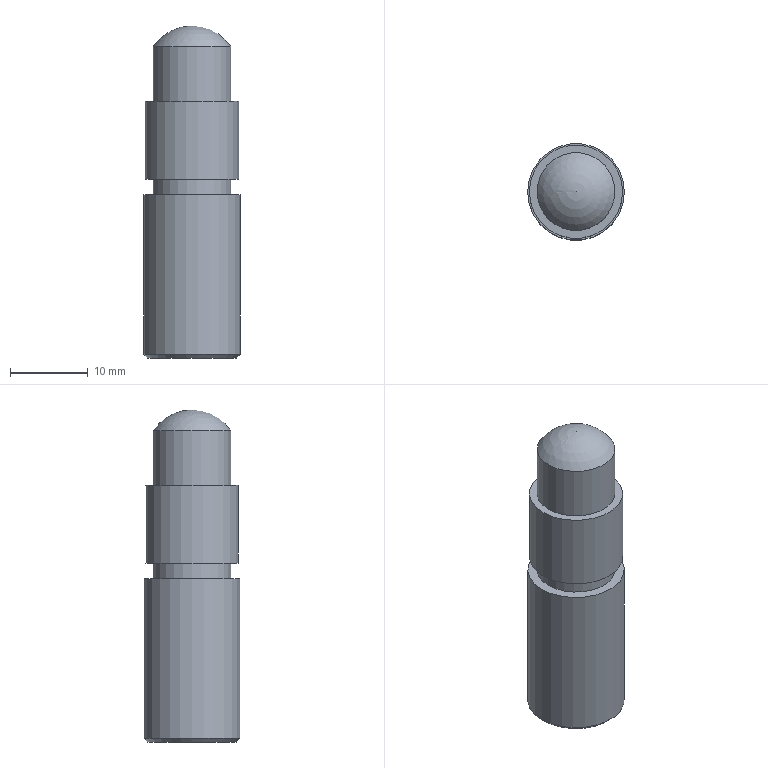Component | NX | EJECTOR_PIN | 1 solid | 10 faces | box 12.42 x 12.42 x 42.68 mm | volume 4494 mm3 | plane 4 | cylinder 4 | sphere 1 | cone 1 | commonest cylinder face diameters 10 x2 12.423 x1 12 x1
STEP:
#1=CARTESIAN_POINT('',(0.,0.,0.));
#2=DIRECTION('',(0.,0.,1.));
#3=DIRECTION('',(1.,0.,0.));
#4=AXIS2_PLACEMENT_3D('',#1,#2,#3);
#5=CARTESIAN_POINT('',(12.5,-0.,99.003));
#6=VERTEX_POINT('',#5);
#7=CARTESIAN_POINT('',(7.5,-0.,99.003));
#8=DIRECTION('',(0.,0.,1.));
#9=DIRECTION('',(1.,0.,0.));
#10=AXIS2_PLACEMENT_3D('',#7,#8,#9);
#11=CIRCLE('',#10,5.);
#12=CARTESIAN_POINT('',(7.5,-0.,99.003));
#13=DIRECTION('',(0.,0.,1.));
#14=DIRECTION('',(1.,0.,0.));
#15=AXIS2_PLACEMENT_3D('',#12,#13,#14);
#16=PLANE('',#15);
#17=CARTESIAN_POINT('',(0.,-0.));
#18=DIRECTION('',(1.,0.));
#19=AXIS2_PLACEMENT_2D('',#17,#18);
#20=CIRCLE('',#19,5.);
#21=(GEOMETRIC_REPRESENTATION_CONTEXT(2)PARAMETRIC_REPRESENTATION_CONTEXT()REPRESENTATION_CONTEXT('',''));
#22=DEFINITIONAL_REPRESENTATION('',(#20),#21);
#23=PCURVE('',#16,#22);
#24=CARTESIAN_POINT('',(7.5,-0.,99.003));
#25=DIRECTION('',(0.,0.,1.));
#26=DIRECTION('',(1.,0.,0.));
#27=AXIS2_PLACEMENT_3D('',#24,#25,#26);
#28=CYLINDRICAL_SURFACE('',#27,5.);
#29=CARTESIAN_POINT('',(0.,0.));
#30=DIRECTION('',(1.,0.));
#31=VECTOR('',#30,1.);
#32=LINE('',#29,#31);
#33=(GEOMETRIC_REPRESENTATION_CONTEXT(2)PARAMETRIC_REPRESENTATION_CONTEXT()REPRESENTATION_CONTEXT('',''));
#34=DEFINITIONAL_REPRESENTATION('',(#32),#33);
#35=PCURVE('',#28,#34);
#36=SURFACE_CURVE('',#11,(#23,#35),.PCURVE_S1.);
#37=EDGE_CURVE('',#6,#6,#36,.T.);
#38=ORIENTED_EDGE('',*,*,#37,.F.);
#39=EDGE_LOOP('',(#38));
#40=FACE_BOUND('',#39,.T.);
#41=CARTESIAN_POINT('',(13.712,-0.,99.003));
#42=VERTEX_POINT('',#41);
#43=CARTESIAN_POINT('',(7.5,-0.,99.003));
#44=DIRECTION('',(0.,0.,-1.));
#45=DIRECTION('',(1.,0.,0.));
#46=AXIS2_PLACEMENT_3D('',#43,#44,#45);
#47=CIRCLE('',#46,6.212);
#48=CARTESIAN_POINT('',(6.212,0.));
#49=CARTESIAN_POINT('',(6.212,-10.759));
#50=CARTESIAN_POINT('',(-3.106,-5.379));
#51=CARTESIAN_POINT('',(-12.423,-0.));
#52=CARTESIAN_POINT('',(-3.106,5.379));
#53=CARTESIAN_POINT('',(6.212,10.759));
#54=CARTESIAN_POINT('',(6.212,0.));
#55=(BOUNDED_CURVE()B_SPLINE_CURVE(2,(#48,#49,#50,#51,#52,#53,#54),.UNSPECIFIED.,.T.,.F.)B_SPLINE_CURVE_WITH_KNOTS((1,2,2,2,2,1),(-2.094,0.,2.094,4.189,6.283,8.378),.UNSPECIFIED.)CURVE()GEOMETRIC_REPRESENTATION_ITEM()RATIONAL_B_SPLINE_CURVE((1.,0.5,1.,0.5,1.,0.5,1.))REPRESENTATION_ITEM(''));
#56=(GEOMETRIC_REPRESENTATION_CONTEXT(2)PARAMETRIC_REPRESENTATION_CONTEXT()REPRESENTATION_CONTEXT('',''));
#57=DEFINITIONAL_REPRESENTATION('',(#55),#56);
#58=PCURVE('',#16,#57);
#59=CARTESIAN_POINT('',(7.5,-0.,78.003));
#60=DIRECTION('',(0.,0.,1.));
#61=DIRECTION('',(1.,0.,0.));
#62=AXIS2_PLACEMENT_3D('',#59,#60,#61);
#63=CYLINDRICAL_SURFACE('',#62,6.212);
#64=CARTESIAN_POINT('',(6.283,21.));
#65=DIRECTION('',(-1.,0.));
#66=VECTOR('',#65,1.);
#67=LINE('',#64,#66);
#68=(GEOMETRIC_REPRESENTATION_CONTEXT(2)PARAMETRIC_REPRESENTATION_CONTEXT()REPRESENTATION_CONTEXT('',''));
#69=DEFINITIONAL_REPRESENTATION('',(#67),#68);
#70=PCURVE('',#63,#69);
#71=SURFACE_CURVE('',#47,(#58,#70),.PCURVE_S1.);
#72=EDGE_CURVE('',#42,#42,#71,.T.);
#73=ORIENTED_EDGE('',*,*,#72,.F.);
#74=EDGE_LOOP('',(#73));
#75=FACE_BOUND('',#74,.T.);
#76=ADVANCED_FACE('',(#40,#75),#16,.T.);
#77=CARTESIAN_POINT('',(1.788,-0.,78.003));
#78=VERTEX_POINT('',#77);
#79=CARTESIAN_POINT('',(7.5,-0.,78.003));
#80=DIRECTION('',(0.,0.,-1.));
#81=DIRECTION('',(-1.,0.,0.));
#82=AXIS2_PLACEMENT_3D('',#79,#80,#81);
#83=CIRCLE('',#82,5.712);
#84=CARTESIAN_POINT('',(7.5,-0.,78.003));
#85=DIRECTION('',(0.,0.,-1.));
#86=DIRECTION('',(-1.,0.,0.));
#87=AXIS2_PLACEMENT_3D('',#84,#85,#86);
#88=PLANE('',#87);
#89=CARTESIAN_POINT('',(0.,0.));
#90=DIRECTION('',(1.,0.));
#91=AXIS2_PLACEMENT_2D('',#89,#90);
#92=CIRCLE('',#91,5.712);
#93=(GEOMETRIC_REPRESENTATION_CONTEXT(2)PARAMETRIC_REPRESENTATION_CONTEXT()REPRESENTATION_CONTEXT('',''));
#94=DEFINITIONAL_REPRESENTATION('',(#92),#93);
#95=PCURVE('',#88,#94);
#96=CARTESIAN_POINT('',(7.5,-0.,78.503));
#97=DIRECTION('',(0.,0.,1.));
#98=DIRECTION('',(1.,0.,0.));
#99=AXIS2_PLACEMENT_3D('',#96,#97,#98);
#100=CONICAL_SURFACE('',#99,6.212,0.7854);
#101=CARTESIAN_POINT('',(9.425,-0.5));
#102=DIRECTION('',(-1.,0.));
#103=VECTOR('',#102,1.);
#104=LINE('',#101,#103);
#105=(GEOMETRIC_REPRESENTATION_CONTEXT(2)PARAMETRIC_REPRESENTATION_CONTEXT()REPRESENTATION_CONTEXT('',''));
#106=DEFINITIONAL_REPRESENTATION('',(#104),#105);
#107=PCURVE('',#100,#106);
#108=SURFACE_CURVE('',#83,(#95,#107),.PCURVE_S1.);
#109=EDGE_CURVE('',#78,#78,#108,.T.);
#110=ORIENTED_EDGE('',*,*,#109,.T.);
#111=EDGE_LOOP('',(#110));
#112=FACE_BOUND('',#111,.T.);
#113=ADVANCED_FACE('',(#112),#88,.T.);
#114=CARTESIAN_POINT('',(1.288,-0.,78.503));
#115=VERTEX_POINT('',#114);
#116=CARTESIAN_POINT('',(13.712,-0.,78.503));
#117=VERTEX_POINT('',#116);
#118=CARTESIAN_POINT('',(7.5,-0.,78.503));
#119=DIRECTION('',(0.,0.,1.));
#120=DIRECTION('',(-1.,0.,0.));
#121=AXIS2_PLACEMENT_3D('',#118,#119,#120);
#122=CIRCLE('',#121,6.212);
#123=CARTESIAN_POINT('',(3.142,0.5));
#124=DIRECTION('',(1.,0.));
#125=VECTOR('',#124,1.);
#126=LINE('',#123,#125);
#127=(GEOMETRIC_REPRESENTATION_CONTEXT(2)PARAMETRIC_REPRESENTATION_CONTEXT()REPRESENTATION_CONTEXT('',''));
#128=DEFINITIONAL_REPRESENTATION('',(#126),#127);
#129=PCURVE('',#63,#128);
#130=CARTESIAN_POINT('',(3.142,0.));
#131=DIRECTION('',(1.,-0.));
#132=VECTOR('',#131,1.);
#133=LINE('',#130,#132);
#134=(GEOMETRIC_REPRESENTATION_CONTEXT(2)PARAMETRIC_REPRESENTATION_CONTEXT()REPRESENTATION_CONTEXT('',''));
#135=DEFINITIONAL_REPRESENTATION('',(#133),#134);
#136=PCURVE('',#100,#135);
#137=SURFACE_CURVE('',#122,(#129,#136),.PCURVE_S1.);
#138=EDGE_CURVE('',#115,#117,#137,.T.);
#139=ORIENTED_EDGE('',*,*,#138,.T.);
#140=CARTESIAN_POINT('',(13.712,-0.,78.503));
#141=CARTESIAN_POINT('',(13.712,-0.,99.003));
#142=B_SPLINE_CURVE_WITH_KNOTS('',1,(#140,#141),.UNSPECIFIED.,.F.,.F.,(2,2),(0.5,21.),.PIECEWISE_BEZIER_KNOTS.);
#143=CARTESIAN_POINT('',(6.283,0.));
#144=DIRECTION('',(0.,1.));
#145=VECTOR('',#144,1.);
#146=LINE('',#143,#145);
#147=(GEOMETRIC_REPRESENTATION_CONTEXT(2)PARAMETRIC_REPRESENTATION_CONTEXT()REPRESENTATION_CONTEXT('',''));
#148=DEFINITIONAL_REPRESENTATION('',(#146),#147);
#149=PCURVE('',#63,#148);
#150=CARTESIAN_POINT('',(0.,0.));
#151=DIRECTION('',(0.,1.));
#152=VECTOR('',#151,1.);
#153=LINE('',#150,#152);
#154=(GEOMETRIC_REPRESENTATION_CONTEXT(2)PARAMETRIC_REPRESENTATION_CONTEXT()REPRESENTATION_CONTEXT('',''));
#155=DEFINITIONAL_REPRESENTATION('',(#153),#154);
#156=PCURVE('',#63,#155);
#157=SEAM_CURVE('',#142,(#149,#156),.PCURVE_S1.);
#158=EDGE_CURVE('',#117,#42,#157,.T.);
#159=ORIENTED_EDGE('',*,*,#158,.T.);
#160=ORIENTED_EDGE('',*,*,#72,.T.);
#161=ORIENTED_EDGE('',*,*,#158,.F.);
#162=CARTESIAN_POINT('',(7.5,-0.,78.503));
#163=DIRECTION('',(0.,0.,1.));
#164=DIRECTION('',(-1.,0.,0.));
#165=AXIS2_PLACEMENT_3D('',#162,#163,#164);
#166=CIRCLE('',#165,6.212);
#167=CARTESIAN_POINT('',(-3.142,0.5));
#168=DIRECTION('',(1.,0.));
#169=VECTOR('',#168,1.);
#170=LINE('',#167,#169);
#171=(GEOMETRIC_REPRESENTATION_CONTEXT(2)PARAMETRIC_REPRESENTATION_CONTEXT()REPRESENTATION_CONTEXT('',''));
#172=DEFINITIONAL_REPRESENTATION('',(#170),#171);
#173=PCURVE('',#63,#172);
#174=CARTESIAN_POINT('',(3.142,-0.));
#175=DIRECTION('',(1.,0.));
#176=VECTOR('',#175,1.);
#177=LINE('',#174,#176);
#178=(GEOMETRIC_REPRESENTATION_CONTEXT(2)PARAMETRIC_REPRESENTATION_CONTEXT()REPRESENTATION_CONTEXT('',''));
#179=DEFINITIONAL_REPRESENTATION('',(#177),#178);
#180=PCURVE('',#100,#179);
#181=SURFACE_CURVE('',#166,(#173,#180),.PCURVE_S1.);
#182=EDGE_CURVE('',#117,#115,#181,.T.);
#183=ORIENTED_EDGE('',*,*,#182,.T.);
#184=EDGE_LOOP('',(#139,#159,#160,#161,#183));
#185=FACE_BOUND('',#184,.T.);
#186=ADVANCED_FACE('',(#185),#63,.T.);
#187=CARTESIAN_POINT('',(12.5,-0.,101.003));
#188=VERTEX_POINT('',#187);
#189=CARTESIAN_POINT('',(7.5,-0.,101.003));
#190=DIRECTION('',(0.,0.,1.));
#191=DIRECTION('',(1.,0.,0.));
#192=AXIS2_PLACEMENT_3D('',#189,#190,#191);
#193=CIRCLE('',#192,5.);
#194=CARTESIAN_POINT('',(0.,2.));
#195=DIRECTION('',(1.,0.));
#196=VECTOR('',#195,1.);
#197=LINE('',#194,#196);
#198=(GEOMETRIC_REPRESENTATION_CONTEXT(2)PARAMETRIC_REPRESENTATION_CONTEXT()REPRESENTATION_CONTEXT('',''));
#199=DEFINITIONAL_REPRESENTATION('',(#197),#198);
#200=PCURVE('',#28,#199);
#201=CARTESIAN_POINT('',(7.5,-0.,101.003));
#202=DIRECTION('',(0.,0.,-1.));
#203=DIRECTION('',(-1.,0.,0.));
#204=AXIS2_PLACEMENT_3D('',#201,#202,#203);
#205=PLANE('',#204);
#206=CARTESIAN_POINT('',(-5.,-0.));
#207=CARTESIAN_POINT('',(-5.,8.66));
#208=CARTESIAN_POINT('',(2.5,4.33));
#209=CARTESIAN_POINT('',(10.,0.));
#210=CARTESIAN_POINT('',(2.5,-4.33));
#211=CARTESIAN_POINT('',(-5.,-8.66));
#212=CARTESIAN_POINT('',(-5.,-0.));
#213=(BOUNDED_CURVE()B_SPLINE_CURVE(2,(#206,#207,#208,#209,#210,#211,#212),.UNSPECIFIED.,.T.,.F.)B_SPLINE_CURVE_WITH_KNOTS((1,2,2,2,2,1),(-2.094,0.,2.094,4.189,6.283,8.378),.UNSPECIFIED.)CURVE()GEOMETRIC_REPRESENTATION_ITEM()RATIONAL_B_SPLINE_CURVE((1.,0.5,1.,0.5,1.,0.5,1.))REPRESENTATION_ITEM(''));
#214=(GEOMETRIC_REPRESENTATION_CONTEXT(2)PARAMETRIC_REPRESENTATION_CONTEXT()REPRESENTATION_CONTEXT('',''));
#215=DEFINITIONAL_REPRESENTATION('',(#213),#214);
#216=PCURVE('',#205,#215);
#217=SURFACE_CURVE('',#193,(#200,#216),.PCURVE_S1.);
#218=EDGE_CURVE('',#188,#188,#217,.T.);
#219=ORIENTED_EDGE('',*,*,#218,.F.);
#220=CARTESIAN_POINT('',(12.5,-0.,99.003));
#221=CARTESIAN_POINT('',(12.5,-0.,101.003));
#222=B_SPLINE_CURVE_WITH_KNOTS('',1,(#220,#221),.UNSPECIFIED.,.F.,.F.,(2,2),(0.,2.),.PIECEWISE_BEZIER_KNOTS.);
#223=CARTESIAN_POINT('',(0.,0.));
#224=DIRECTION('',(0.,1.));
#225=VECTOR('',#224,1.);
#226=LINE('',#223,#225);
#227=(GEOMETRIC_REPRESENTATION_CONTEXT(2)PARAMETRIC_REPRESENTATION_CONTEXT()REPRESENTATION_CONTEXT('',''));
#228=DEFINITIONAL_REPRESENTATION('',(#226),#227);
#229=PCURVE('',#28,#228);
#230=CARTESIAN_POINT('',(6.283,0.));
#231=DIRECTION('',(0.,1.));
#232=VECTOR('',#231,1.);
#233=LINE('',#230,#232);
#234=(GEOMETRIC_REPRESENTATION_CONTEXT(2)PARAMETRIC_REPRESENTATION_CONTEXT()REPRESENTATION_CONTEXT('',''));
#235=DEFINITIONAL_REPRESENTATION('',(#233),#234);
#236=PCURVE('',#28,#235);
#237=SEAM_CURVE('',#222,(#229,#236),.PCURVE_S1.);
#238=EDGE_CURVE('',#6,#188,#237,.T.);
#239=ORIENTED_EDGE('',*,*,#238,.F.);
#240=ORIENTED_EDGE('',*,*,#37,.T.);
#241=ORIENTED_EDGE('',*,*,#238,.T.);
#242=EDGE_LOOP('',(#219,#239,#240,#241));
#243=FACE_BOUND('',#242,.T.);
#244=ADVANCED_FACE('',(#243),#28,.T.);
#245=CARTESIAN_POINT('',(12.5,-0.,111.003));
#246=VERTEX_POINT('',#245);
#247=CARTESIAN_POINT('',(7.5,-0.,111.003));
#248=DIRECTION('',(0.,0.,1.));
#249=DIRECTION('',(1.,0.,0.));
#250=AXIS2_PLACEMENT_3D('',#247,#248,#249);
#251=CIRCLE('',#250,5.);
#252=CARTESIAN_POINT('',(7.5,-0.,111.003));
#253=DIRECTION('',(0.,0.,1.));
#254=DIRECTION('',(1.,0.,0.));
#255=AXIS2_PLACEMENT_3D('',#252,#253,#254);
#256=PLANE('',#255);
#257=CARTESIAN_POINT('',(0.,0.));
#258=DIRECTION('',(1.,0.));
#259=AXIS2_PLACEMENT_2D('',#257,#258);
#260=CIRCLE('',#259,5.);
#261=(GEOMETRIC_REPRESENTATION_CONTEXT(2)PARAMETRIC_REPRESENTATION_CONTEXT()REPRESENTATION_CONTEXT('',''));
#262=DEFINITIONAL_REPRESENTATION('',(#260),#261);
#263=PCURVE('',#256,#262);
#264=CARTESIAN_POINT('',(7.5,-0.,111.003));
#265=DIRECTION('',(0.,0.,1.));
#266=DIRECTION('',(1.,0.,0.));
#267=AXIS2_PLACEMENT_3D('',#264,#265,#266);
#268=CYLINDRICAL_SURFACE('',#267,5.);
#269=CARTESIAN_POINT('',(0.,0.));
#270=DIRECTION('',(1.,0.));
#271=VECTOR('',#270,1.);
#272=LINE('',#269,#271);
#273=(GEOMETRIC_REPRESENTATION_CONTEXT(2)PARAMETRIC_REPRESENTATION_CONTEXT()REPRESENTATION_CONTEXT('',''));
#274=DEFINITIONAL_REPRESENTATION('',(#272),#273);
#275=PCURVE('',#268,#274);
#276=SURFACE_CURVE('',#251,(#263,#275),.PCURVE_S1.);
#277=EDGE_CURVE('',#246,#246,#276,.T.);
#278=ORIENTED_EDGE('',*,*,#277,.F.);
#279=EDGE_LOOP('',(#278));
#280=FACE_BOUND('',#279,.T.);
#281=CARTESIAN_POINT('',(13.5,-0.,111.003));
#282=VERTEX_POINT('',#281);
#283=CARTESIAN_POINT('',(7.5,-0.,111.003));
#284=DIRECTION('',(0.,0.,1.));
#285=DIRECTION('',(1.,0.,0.));
#286=AXIS2_PLACEMENT_3D('',#283,#284,#285);
#287=CIRCLE('',#286,6.);
#288=CARTESIAN_POINT('',(0.,0.));
#289=DIRECTION('',(1.,0.));
#290=AXIS2_PLACEMENT_2D('',#288,#289);
#291=CIRCLE('',#290,6.);
#292=(GEOMETRIC_REPRESENTATION_CONTEXT(2)PARAMETRIC_REPRESENTATION_CONTEXT()REPRESENTATION_CONTEXT('',''));
#293=DEFINITIONAL_REPRESENTATION('',(#291),#292);
#294=PCURVE('',#256,#293);
#295=CARTESIAN_POINT('',(7.5,-0.,101.003));
#296=DIRECTION('',(0.,0.,1.));
#297=DIRECTION('',(1.,0.,0.));
#298=AXIS2_PLACEMENT_3D('',#295,#296,#297);
#299=CYLINDRICAL_SURFACE('',#298,6.);
#300=CARTESIAN_POINT('',(0.,10.));
#301=DIRECTION('',(1.,0.));
#302=VECTOR('',#301,1.);
#303=LINE('',#300,#302);
#304=(GEOMETRIC_REPRESENTATION_CONTEXT(2)PARAMETRIC_REPRESENTATION_CONTEXT()REPRESENTATION_CONTEXT('',''));
#305=DEFINITIONAL_REPRESENTATION('',(#303),#304);
#306=PCURVE('',#299,#305);
#307=SURFACE_CURVE('',#287,(#294,#306),.PCURVE_S1.);
#308=EDGE_CURVE('',#282,#282,#307,.T.);
#309=ORIENTED_EDGE('',*,*,#308,.T.);
#310=EDGE_LOOP('',(#309));
#311=FACE_BOUND('',#310,.T.);
#312=ADVANCED_FACE('',(#280,#311),#256,.T.);
#313=ORIENTED_EDGE('',*,*,#218,.T.);
#314=EDGE_LOOP('',(#313));
#315=FACE_BOUND('',#314,.T.);
#316=CARTESIAN_POINT('',(13.5,-0.,101.003));
#317=VERTEX_POINT('',#316);
#318=CARTESIAN_POINT('',(7.5,-0.,101.003));
#319=DIRECTION('',(0.,0.,1.));
#320=DIRECTION('',(1.,0.,0.));
#321=AXIS2_PLACEMENT_3D('',#318,#319,#320);
#322=CIRCLE('',#321,6.);
#323=CARTESIAN_POINT('',(-6.,0.));
#324=CARTESIAN_POINT('',(-6.,10.392));
#325=CARTESIAN_POINT('',(3.,5.196));
#326=CARTESIAN_POINT('',(12.,0.));
#327=CARTESIAN_POINT('',(3.,-5.196));
#328=CARTESIAN_POINT('',(-6.,-10.392));
#329=CARTESIAN_POINT('',(-6.,0.));
#330=(BOUNDED_CURVE()B_SPLINE_CURVE(2,(#323,#324,#325,#326,#327,#328,#329),.UNSPECIFIED.,.T.,.F.)B_SPLINE_CURVE_WITH_KNOTS((1,2,2,2,2,1),(-2.094,0.,2.094,4.189,6.283,8.378),.UNSPECIFIED.)CURVE()GEOMETRIC_REPRESENTATION_ITEM()RATIONAL_B_SPLINE_CURVE((1.,0.5,1.,0.5,1.,0.5,1.))REPRESENTATION_ITEM(''));
#331=(GEOMETRIC_REPRESENTATION_CONTEXT(2)PARAMETRIC_REPRESENTATION_CONTEXT()REPRESENTATION_CONTEXT('',''));
#332=DEFINITIONAL_REPRESENTATION('',(#330),#331);
#333=PCURVE('',#205,#332);
#334=CARTESIAN_POINT('',(0.,0.));
#335=DIRECTION('',(1.,0.));
#336=VECTOR('',#335,1.);
#337=LINE('',#334,#336);
#338=(GEOMETRIC_REPRESENTATION_CONTEXT(2)PARAMETRIC_REPRESENTATION_CONTEXT()REPRESENTATION_CONTEXT('',''));
#339=DEFINITIONAL_REPRESENTATION('',(#337),#338);
#340=PCURVE('',#299,#339);
#341=SURFACE_CURVE('',#322,(#333,#340),.PCURVE_S1.);
#342=EDGE_CURVE('',#317,#317,#341,.T.);
#343=ORIENTED_EDGE('',*,*,#342,.F.);
#344=EDGE_LOOP('',(#343));
#345=FACE_BOUND('',#344,.T.);
#346=ADVANCED_FACE('',(#315,#345),#205,.T.);
#347=ORIENTED_EDGE('',*,*,#308,.F.);
#348=CARTESIAN_POINT('',(13.5,-0.,101.003));
#349=CARTESIAN_POINT('',(13.5,-0.,111.003));
#350=B_SPLINE_CURVE_WITH_KNOTS('',1,(#348,#349),.UNSPECIFIED.,.F.,.F.,(2,2),(0.,10.),.PIECEWISE_BEZIER_KNOTS.);
#351=CARTESIAN_POINT('',(0.,0.));
#352=DIRECTION('',(0.,1.));
#353=VECTOR('',#352,1.);
#354=LINE('',#351,#353);
#355=(GEOMETRIC_REPRESENTATION_CONTEXT(2)PARAMETRIC_REPRESENTATION_CONTEXT()REPRESENTATION_CONTEXT('',''));
#356=DEFINITIONAL_REPRESENTATION('',(#354),#355);
#357=PCURVE('',#299,#356);
#358=CARTESIAN_POINT('',(6.283,0.));
#359=DIRECTION('',(0.,1.));
#360=VECTOR('',#359,1.);
#361=LINE('',#358,#360);
#362=(GEOMETRIC_REPRESENTATION_CONTEXT(2)PARAMETRIC_REPRESENTATION_CONTEXT()REPRESENTATION_CONTEXT('',''));
#363=DEFINITIONAL_REPRESENTATION('',(#361),#362);
#364=PCURVE('',#299,#363);
#365=SEAM_CURVE('',#350,(#357,#364),.PCURVE_S1.);
#366=EDGE_CURVE('',#317,#282,#365,.T.);
#367=ORIENTED_EDGE('',*,*,#366,.F.);
#368=ORIENTED_EDGE('',*,*,#342,.T.);
#369=ORIENTED_EDGE('',*,*,#366,.T.);
#370=EDGE_LOOP('',(#347,#367,#368,#369));
#371=FACE_BOUND('',#370,.T.);
#372=ADVANCED_FACE('',(#371),#299,.T.);
#373=CARTESIAN_POINT('',(12.5,-0.,118.003));
#374=VERTEX_POINT('',#373);
#375=CARTESIAN_POINT('',(2.5,-0.,118.003));
#376=VERTEX_POINT('',#375);
#377=CARTESIAN_POINT('',(7.5,-0.,118.003));
#378=DIRECTION('',(0.,0.,1.));
#379=DIRECTION('',(1.,0.,0.));
#380=AXIS2_PLACEMENT_3D('',#377,#378,#379);
#381=CIRCLE('',#380,5.);
#382=CARTESIAN_POINT('',(0.,7.));
#383=DIRECTION('',(1.,0.));
#384=VECTOR('',#383,1.);
#385=LINE('',#382,#384);
#386=(GEOMETRIC_REPRESENTATION_CONTEXT(2)PARAMETRIC_REPRESENTATION_CONTEXT()REPRESENTATION_CONTEXT('',''));
#387=DEFINITIONAL_REPRESENTATION('',(#385),#386);
#388=PCURVE('',#268,#387);
#389=CARTESIAN_POINT('',(7.5,-0.,114.687));
#390=DIRECTION('',(0.,0.,1.));
#391=DIRECTION('',(-1.,0.,0.));
#392=AXIS2_PLACEMENT_3D('',#389,#390,#391);
#393=SPHERICAL_SURFACE('',#392,6.);
#394=CARTESIAN_POINT('',(3.142,0.5857));
#395=CARTESIAN_POINT('',(3.237,0.5857));
#396=CARTESIAN_POINT('',(3.427,0.5857));
#397=CARTESIAN_POINT('',(3.713,0.5857));
#398=CARTESIAN_POINT('',(3.998,0.5857));
#399=CARTESIAN_POINT('',(4.284,0.5857));
#400=CARTESIAN_POINT('',(4.57,0.5857));
#401=CARTESIAN_POINT('',(4.855,0.5857));
#402=CARTESIAN_POINT('',(5.141,0.5857));
#403=CARTESIAN_POINT('',(5.426,0.5857));
#404=CARTESIAN_POINT('',(5.712,0.5857));
#405=CARTESIAN_POINT('',(5.998,0.5857));
#406=CARTESIAN_POINT('',(6.283,0.5857));
#407=CARTESIAN_POINT('',(6.569,0.5857));
#408=CARTESIAN_POINT('',(6.854,0.5857));
#409=CARTESIAN_POINT('',(7.14,0.5857));
#410=CARTESIAN_POINT('',(7.426,0.5857));
#411=CARTESIAN_POINT('',(7.711,0.5857));
#412=CARTESIAN_POINT('',(7.997,0.5857));
#413=CARTESIAN_POINT('',(8.282,0.5857));
#414=CARTESIAN_POINT('',(8.568,0.5857));
#415=CARTESIAN_POINT('',(8.854,0.5857));
#416=CARTESIAN_POINT('',(9.139,0.5857));
#417=CARTESIAN_POINT('',(9.33,0.5857));
#418=CARTESIAN_POINT('',(9.425,0.5857));
#419=B_SPLINE_CURVE_WITH_KNOTS('',3,(#394,#395,#396,#397,#398,#399,#400,#401,#402,#403,#404,#405,#406,#407,#408,#409,#410,#411,#412,#413,#414,#415,#416,#417,#418),.UNSPECIFIED.,.F.,.F.,(4,1,1,1,1,1,1,1,1,1,1,1,1,1,1,1,1,1,1,1,1,1,4),(0.,0.2856,0.5712,0.8568,1.142,1.428,1.714,1.999,2.285,2.57,2.856,3.142,3.427,3.713,3.998,4.284,4.57,4.855,5.141,5.426,5.712,5.998,6.283),.QUASI_UNIFORM_KNOTS.);
#420=(GEOMETRIC_REPRESENTATION_CONTEXT(2)PARAMETRIC_REPRESENTATION_CONTEXT()REPRESENTATION_CONTEXT('',''));
#421=DEFINITIONAL_REPRESENTATION('',(#419),#420);
#422=PCURVE('',#393,#421);
#423=SURFACE_CURVE('',#381,(#388,#422),.PCURVE_S1.);
#424=EDGE_CURVE('',#374,#376,#423,.T.);
#425=ORIENTED_EDGE('',*,*,#424,.F.);
#426=CARTESIAN_POINT('',(12.5,-0.,111.003));
#427=CARTESIAN_POINT('',(12.5,-0.,118.003));
#428=B_SPLINE_CURVE_WITH_KNOTS('',1,(#426,#427),.UNSPECIFIED.,.F.,.F.,(2,2),(0.,7.),.PIECEWISE_BEZIER_KNOTS.);
#429=CARTESIAN_POINT('',(0.,0.));
#430=DIRECTION('',(0.,1.));
#431=VECTOR('',#430,1.);
#432=LINE('',#429,#431);
#433=(GEOMETRIC_REPRESENTATION_CONTEXT(2)PARAMETRIC_REPRESENTATION_CONTEXT()REPRESENTATION_CONTEXT('',''));
#434=DEFINITIONAL_REPRESENTATION('',(#432),#433);
#435=PCURVE('',#268,#434);
#436=CARTESIAN_POINT('',(6.283,0.));
#437=DIRECTION('',(0.,1.));
#438=VECTOR('',#437,1.);
#439=LINE('',#436,#438);
#440=(GEOMETRIC_REPRESENTATION_CONTEXT(2)PARAMETRIC_REPRESENTATION_CONTEXT()REPRESENTATION_CONTEXT('',''));
#441=DEFINITIONAL_REPRESENTATION('',(#439),#440);
#442=PCURVE('',#268,#441);
#443=SEAM_CURVE('',#428,(#435,#442),.PCURVE_S1.);
#444=EDGE_CURVE('',#246,#374,#443,.T.);
#445=ORIENTED_EDGE('',*,*,#444,.F.);
#446=ORIENTED_EDGE('',*,*,#277,.T.);
#447=ORIENTED_EDGE('',*,*,#444,.T.);
#448=CARTESIAN_POINT('',(7.5,-0.,118.003));
#449=DIRECTION('',(0.,0.,1.));
#450=DIRECTION('',(1.,0.,0.));
#451=AXIS2_PLACEMENT_3D('',#448,#449,#450);
#452=CIRCLE('',#451,5.);
#453=CARTESIAN_POINT('',(0.,7.));
#454=DIRECTION('',(1.,0.));
#455=VECTOR('',#454,1.);
#456=LINE('',#453,#455);
#457=(GEOMETRIC_REPRESENTATION_CONTEXT(2)PARAMETRIC_REPRESENTATION_CONTEXT()REPRESENTATION_CONTEXT('',''));
#458=DEFINITIONAL_REPRESENTATION('',(#456),#457);
#459=PCURVE('',#268,#458);
#460=CARTESIAN_POINT('',(-3.142,0.5857));
#461=CARTESIAN_POINT('',(-3.046,0.5857));
#462=CARTESIAN_POINT('',(-2.856,0.5857));
#463=CARTESIAN_POINT('',(-2.57,0.5857));
#464=CARTESIAN_POINT('',(-2.285,0.5857));
#465=CARTESIAN_POINT('',(-1.999,0.5857));
#466=CARTESIAN_POINT('',(-1.714,0.5857));
#467=CARTESIAN_POINT('',(-1.428,0.5857));
#468=CARTESIAN_POINT('',(-1.142,0.5857));
#469=CARTESIAN_POINT('',(-0.8568,0.5857));
#470=CARTESIAN_POINT('',(-0.5712,0.5857));
#471=CARTESIAN_POINT('',(-0.2856,0.5857));
#472=CARTESIAN_POINT('',(0.,0.5857));
#473=CARTESIAN_POINT('',(0.2856,0.5857));
#474=CARTESIAN_POINT('',(0.5712,0.5857));
#475=CARTESIAN_POINT('',(0.8568,0.5857));
#476=CARTESIAN_POINT('',(1.142,0.5857));
#477=CARTESIAN_POINT('',(1.428,0.5857));
#478=CARTESIAN_POINT('',(1.714,0.5857));
#479=CARTESIAN_POINT('',(1.999,0.5857));
#480=CARTESIAN_POINT('',(2.285,0.5857));
#481=CARTESIAN_POINT('',(2.57,0.5857));
#482=CARTESIAN_POINT('',(2.856,0.5857));
#483=CARTESIAN_POINT('',(3.046,0.5857));
#484=CARTESIAN_POINT('',(3.142,0.5857));
#485=B_SPLINE_CURVE_WITH_KNOTS('',3,(#460,#461,#462,#463,#464,#465,#466,#467,#468,#469,#470,#471,#472,#473,#474,#475,#476,#477,#478,#479,#480,#481,#482,#483,#484),.UNSPECIFIED.,.F.,.F.,(4,1,1,1,1,1,1,1,1,1,1,1,1,1,1,1,1,1,1,1,1,1,4),(0.,0.2856,0.5712,0.8568,1.142,1.428,1.714,1.999,2.285,2.57,2.856,3.142,3.427,3.713,3.998,4.284,4.57,4.855,5.141,5.426,5.712,5.998,6.283),.QUASI_UNIFORM_KNOTS.);
#486=(GEOMETRIC_REPRESENTATION_CONTEXT(2)PARAMETRIC_REPRESENTATION_CONTEXT()REPRESENTATION_CONTEXT('',''));
#487=DEFINITIONAL_REPRESENTATION('',(#485),#486);
#488=PCURVE('',#393,#487);
#489=SURFACE_CURVE('',#452,(#459,#488),.PCURVE_S1.);
#490=EDGE_CURVE('',#376,#374,#489,.T.);
#491=ORIENTED_EDGE('',*,*,#490,.F.);
#492=EDGE_LOOP('',(#425,#445,#446,#447,#491));
#493=FACE_BOUND('',#492,.T.);
#494=ADVANCED_FACE('',(#493),#268,.T.);
#495=ORIENTED_EDGE('',*,*,#424,.T.);
#496=CARTESIAN_POINT('',(7.5,-0.,120.687));
#497=VERTEX_POINT('',#496);
#498=CARTESIAN_POINT('',(2.5,-0.,118.003));
#499=CARTESIAN_POINT('',(3.045,-0.,118.824));
#500=CARTESIAN_POINT('',(3.751,-0.,119.538));
#501=CARTESIAN_POINT('',(4.592,-0.,120.104));
#502=CARTESIAN_POINT('',(5.53,-0.,120.492));
#503=CARTESIAN_POINT('',(6.515,-0.,120.687));
#504=CARTESIAN_POINT('',(7.5,-0.,120.687));
#505=B_SPLINE_CURVE_WITH_KNOTS('',6,(#498,#499,#500,#501,#502,#503,#504),.UNSPECIFIED.,.F.,.F.,(7,7),(0.5857,1.571),.PIECEWISE_BEZIER_KNOTS.);
#506=CARTESIAN_POINT('',(6.283,0.));
#507=DIRECTION('',(0.,1.));
#508=VECTOR('',#507,1.);
#509=LINE('',#506,#508);
#510=(GEOMETRIC_REPRESENTATION_CONTEXT(2)PARAMETRIC_REPRESENTATION_CONTEXT()REPRESENTATION_CONTEXT('',''));
#511=DEFINITIONAL_REPRESENTATION('',(#509),#510);
#512=PCURVE('',#393,#511);
#513=CARTESIAN_POINT('',(0.,0.));
#514=DIRECTION('',(0.,1.));
#515=VECTOR('',#514,1.);
#516=LINE('',#513,#515);
#517=(GEOMETRIC_REPRESENTATION_CONTEXT(2)PARAMETRIC_REPRESENTATION_CONTEXT()REPRESENTATION_CONTEXT('',''));
#518=DEFINITIONAL_REPRESENTATION('',(#516),#517);
#519=PCURVE('',#393,#518);
#520=SEAM_CURVE('',#505,(#512,#519),.PCURVE_S1.);
#521=EDGE_CURVE('',#376,#497,#520,.T.);
#522=ORIENTED_EDGE('',*,*,#521,.T.);
#523=ORIENTED_EDGE('',*,*,#521,.F.);
#524=ORIENTED_EDGE('',*,*,#490,.T.);
#525=EDGE_LOOP('',(#495,#522,#523,#524));
#526=FACE_BOUND('',#525,.T.);
#527=ADVANCED_FACE('',(#526),#393,.T.);
#528=ORIENTED_EDGE('',*,*,#109,.F.);
#529=CARTESIAN_POINT('',(1.788,-0.,78.003));
#530=CARTESIAN_POINT('',(1.288,-0.,78.503));
#531=B_SPLINE_CURVE_WITH_KNOTS('',1,(#529,#530),.UNSPECIFIED.,.F.,.F.,(2,2),(-0.7071,0.),.PIECEWISE_BEZIER_KNOTS.);
#532=CARTESIAN_POINT('',(9.425,0.));
#533=DIRECTION('',(0.,1.));
#534=VECTOR('',#533,1.);
#535=LINE('',#532,#534);
#536=(GEOMETRIC_REPRESENTATION_CONTEXT(2)PARAMETRIC_REPRESENTATION_CONTEXT()REPRESENTATION_CONTEXT('',''));
#537=DEFINITIONAL_REPRESENTATION('',(#535),#536);
#538=PCURVE('',#100,#537);
#539=CARTESIAN_POINT('',(3.142,0.));
#540=DIRECTION('',(0.,1.));
#541=VECTOR('',#540,1.);
#542=LINE('',#539,#541);
#543=(GEOMETRIC_REPRESENTATION_CONTEXT(2)PARAMETRIC_REPRESENTATION_CONTEXT()REPRESENTATION_CONTEXT('',''));
#544=DEFINITIONAL_REPRESENTATION('',(#542),#543);
#545=PCURVE('',#100,#544);
#546=SEAM_CURVE('',#531,(#538,#545),.PCURVE_S1.);
#547=EDGE_CURVE('',#78,#115,#546,.T.);
#548=ORIENTED_EDGE('',*,*,#547,.T.);
#549=ORIENTED_EDGE('',*,*,#182,.F.);
#550=ORIENTED_EDGE('',*,*,#138,.F.);
#551=ORIENTED_EDGE('',*,*,#547,.F.);
#552=EDGE_LOOP('',(#528,#548,#549,#550,#551));
#553=FACE_BOUND('',#552,.T.);
#554=ADVANCED_FACE('',(#553),#100,.T.);
#555=CLOSED_SHELL('',(#76,#113,#186,#244,#312,#346,#372,#494,#527,#554));
#556=MANIFOLD_SOLID_BREP('',#555);
#557=(LENGTH_UNIT()NAMED_UNIT(*)SI_UNIT(.MILLI.,.METRE.));
#558=UNCERTAINTY_MEASURE_WITH_UNIT(LENGTH_MEASURE(0.00001),#557,'','');
#559=(NAMED_UNIT(*)PLANE_ANGLE_UNIT()SI_UNIT($,.RADIAN.));
#560=(NAMED_UNIT(*)SI_UNIT($,.STERADIAN.)SOLID_ANGLE_UNIT());
#561=(GEOMETRIC_REPRESENTATION_CONTEXT(3)GLOBAL_UNCERTAINTY_ASSIGNED_CONTEXT((#558))GLOBAL_UNIT_ASSIGNED_CONTEXT((#557,#559,#560))REPRESENTATION_CONTEXT('',''));
#562=ADVANCED_BREP_SHAPE_REPRESENTATION('',(#4,#556),#561);